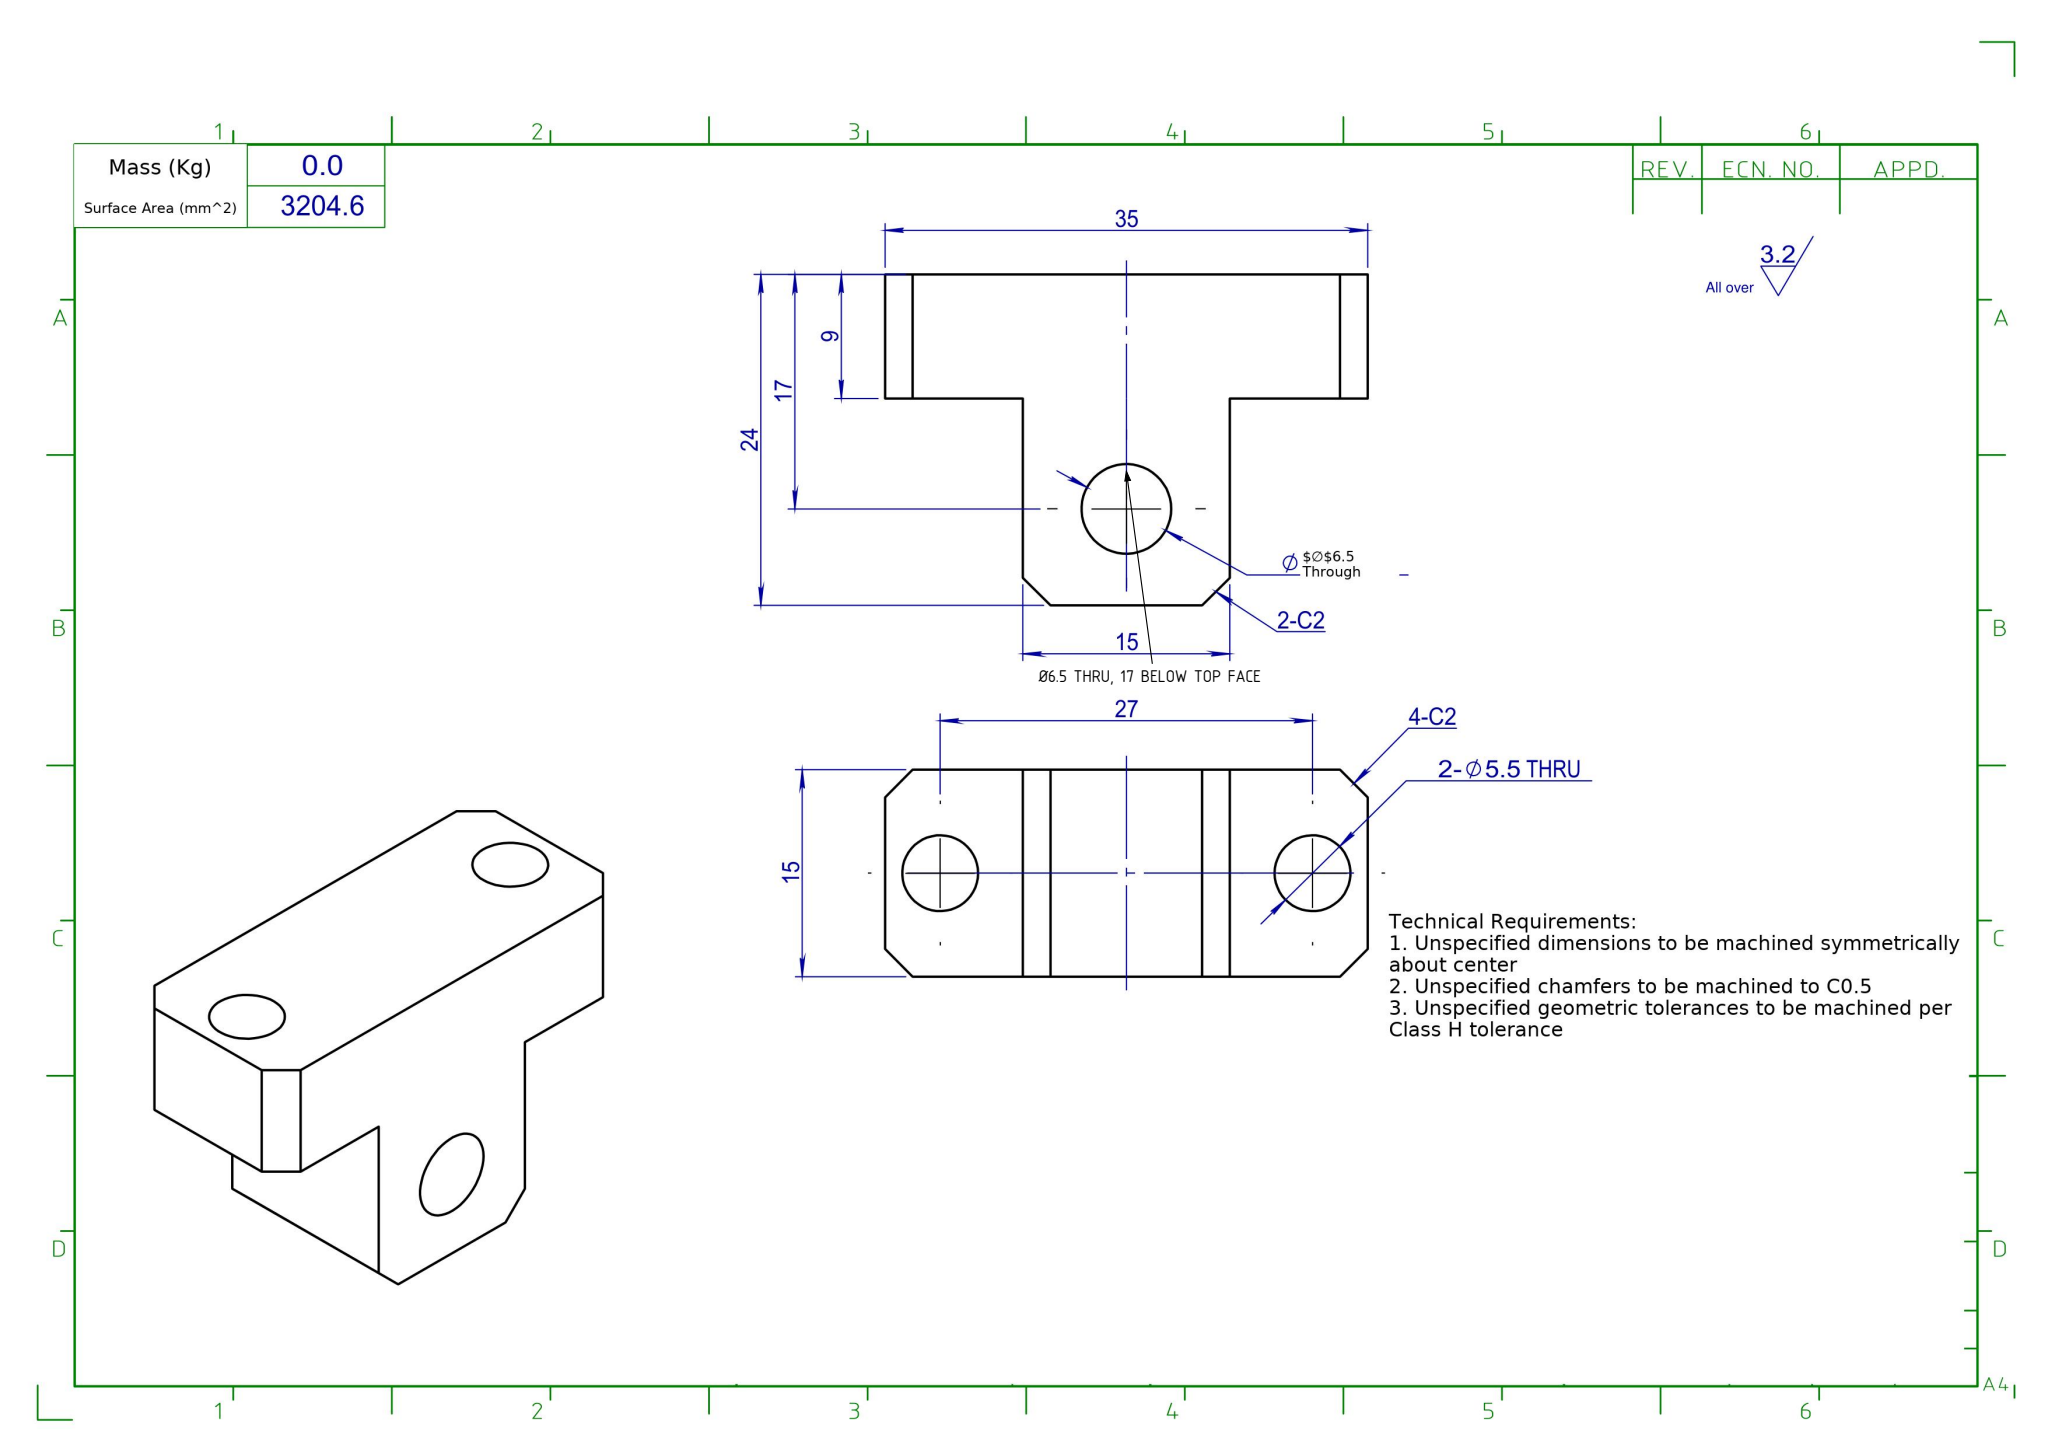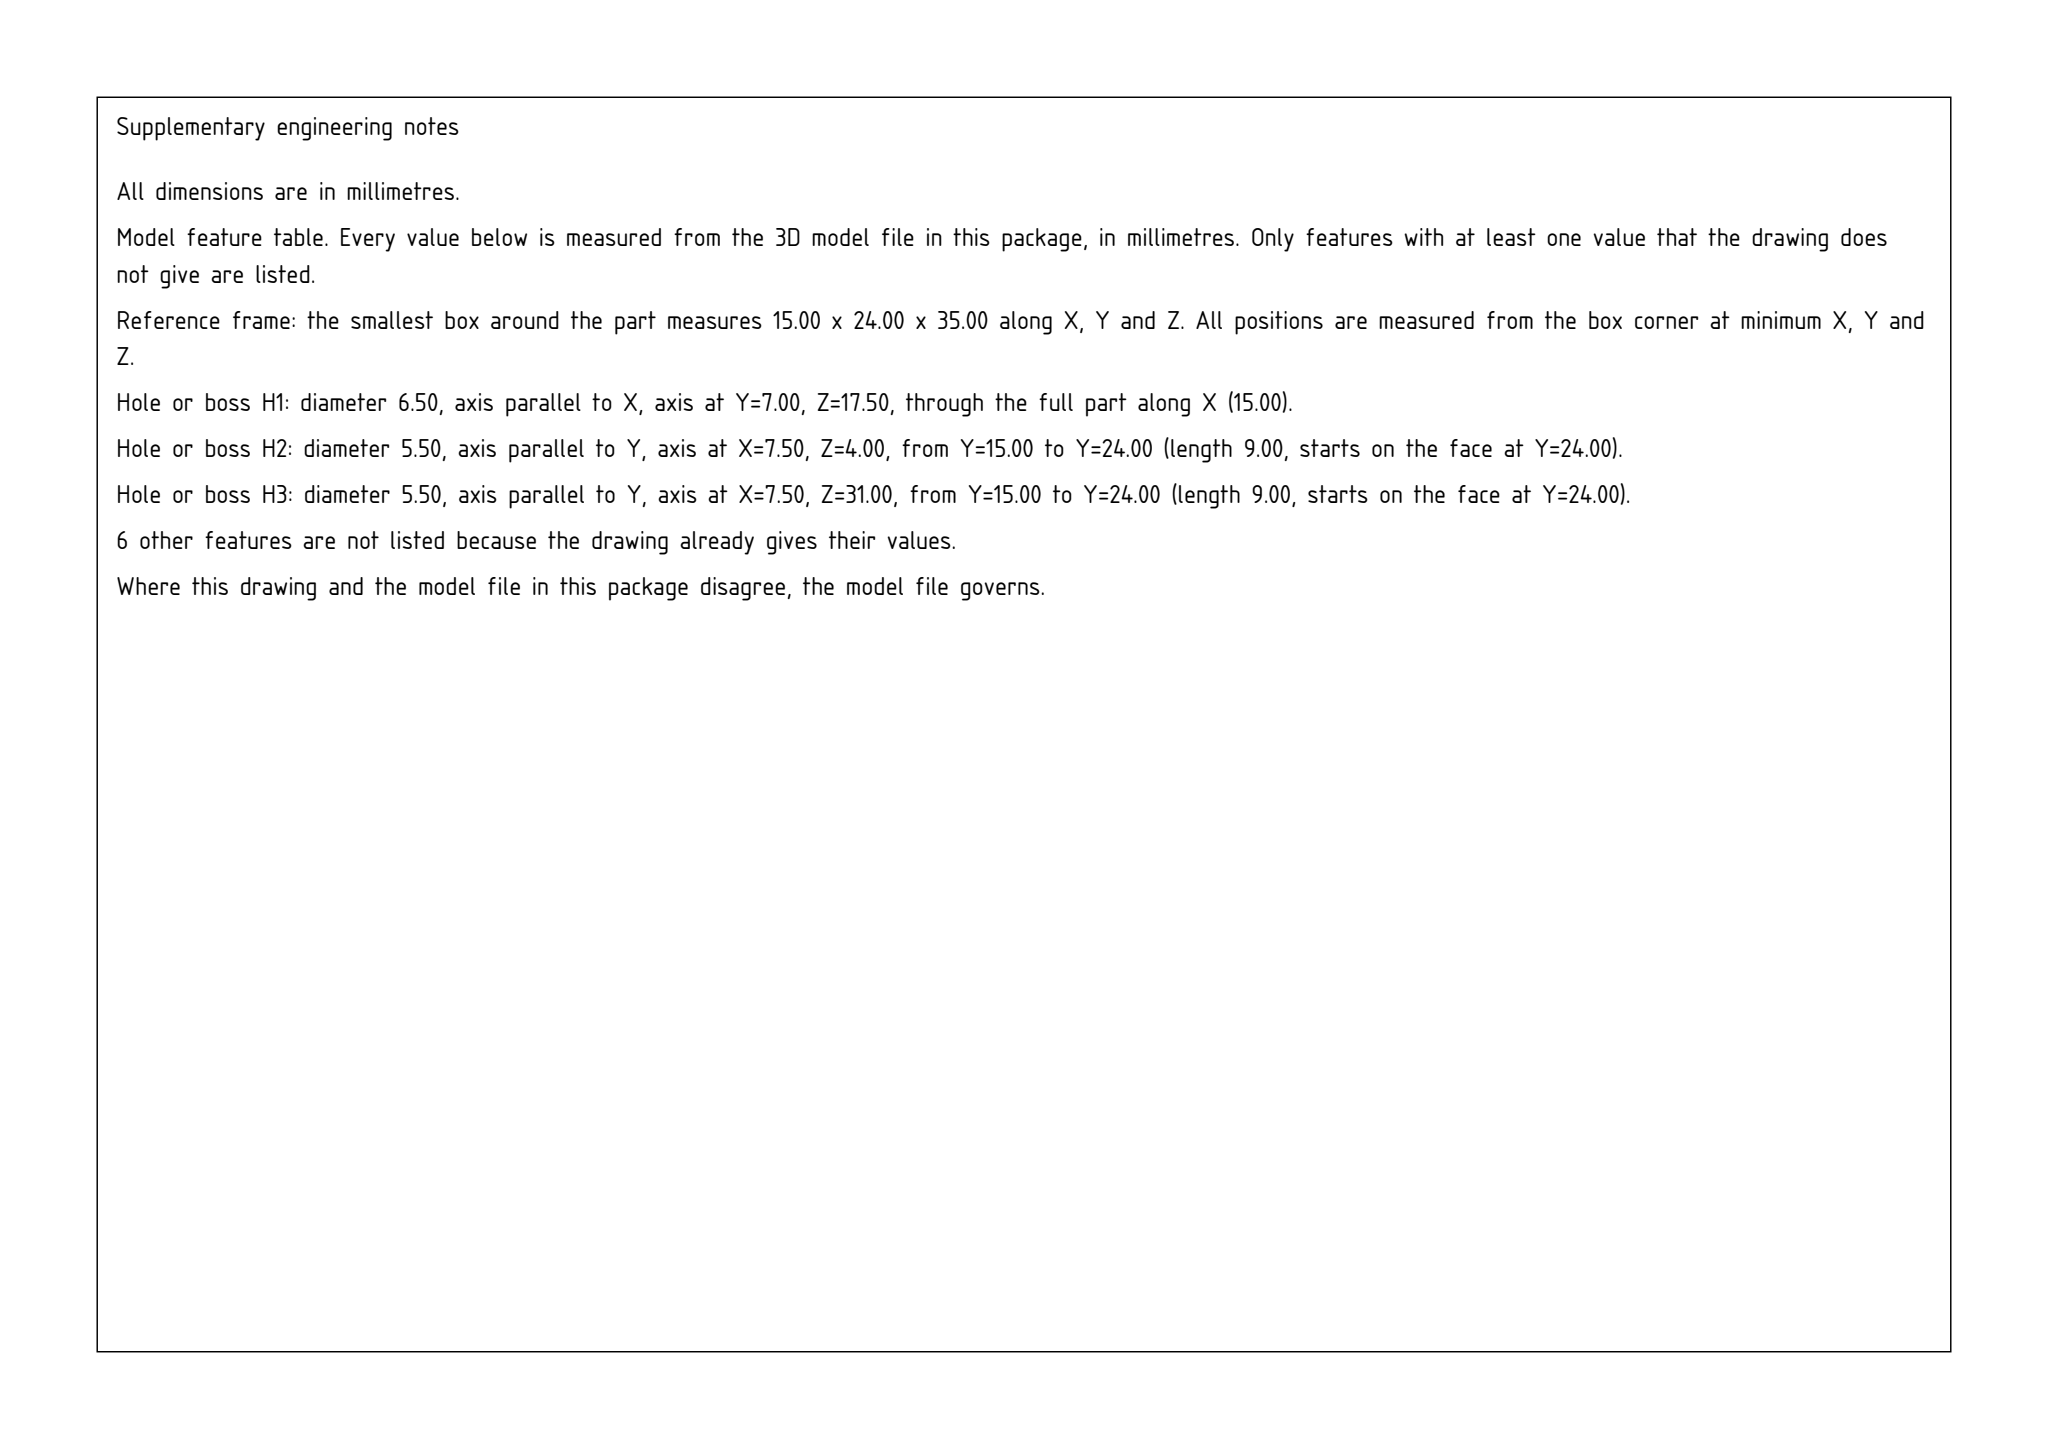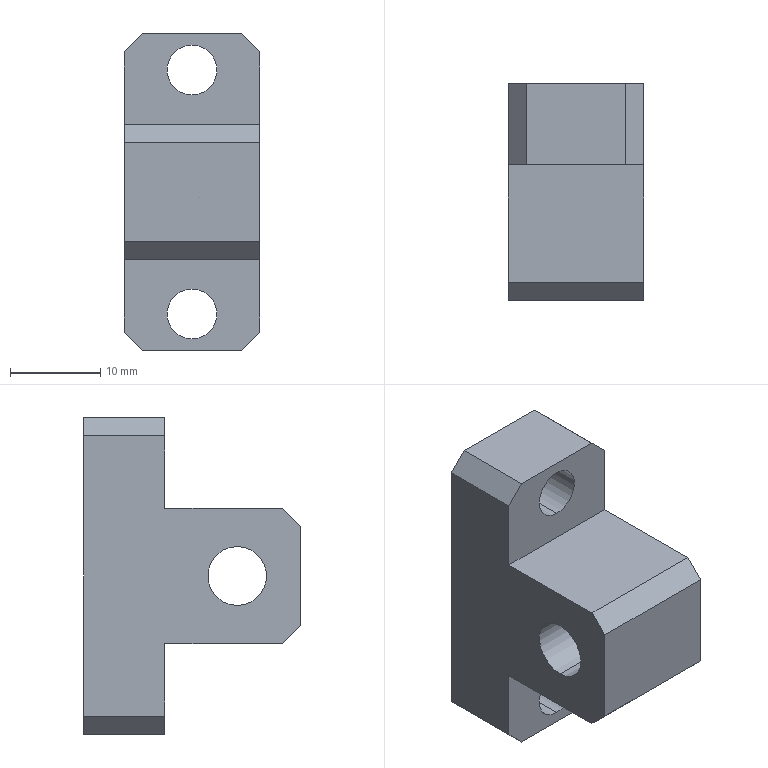Part | SolidWorks | mm | 1 solid | 22 faces | box 15 x 24 x 35 mm | volume 7043 mm3 | plane 16 | cylinder 6 | commonest cylinder face diameters 5.5 x4 6.5 x2
Drawing notes:
Ø6.5 THRU, CTR 17 BELOW TOP FACE, ON VERT CL | from the solid: cylinder hole/bore dia 6.5, axis x, from x=0 to 15 (thru), center y=7.0 of 24 height (=17 below top), z=17.5 = 35/2 centerline
build123d program:
from build123d import *

# Parameters (mm, degrees)
SKETCH1_W          = 15
SKETCH1_H          = 35
EXTRUDE1_DEPTH     = 24
SKETCH2_R          = 3.25
CUT_EXTRUDE1_DEPTH = 34.275
SKETCH3_W          = 15
SKETCH3_H          = 10
CUT_EXTRUDE2_DEPTH = 15
SKETCH4_R          = 2.75
CUT_EXTRUDE3_DEPTH = 25.238
CHAMFER1_SIZE      = 2


with BuildPart() as part:
    # Sketch1 → Extrude1 (new body)
    with BuildSketch(Plane(origin=(0, 0, 0), x_dir=(1, 0, 0), z_dir=(0, 1, 0))):
        Rectangle(SKETCH1_W, SKETCH1_H)
    extrude(amount=EXTRUDE1_DEPTH)

    # Sketch2 → Cut-Extrude1 (cut, through all)
    with BuildSketch(Plane(origin=(7.5, 0, 0), x_dir=(0, 0, -1), z_dir=(1, 0, 0))):
        with Locations((0, 7)):
            Circle(SKETCH2_R)
    extrude(amount=-CUT_EXTRUDE1_DEPTH, mode=Mode.SUBTRACT)

    # Sketch3 → Cut-Extrude2 (cut)
    with BuildSketch(Plane.XZ):
        with Locations((0, 12.5)):
            Rectangle(SKETCH3_W, SKETCH3_H)
        with Locations((0, -12.5)):
            Rectangle(SKETCH3_W, SKETCH3_H)
    extrude(amount=-CUT_EXTRUDE2_DEPTH, mode=Mode.SUBTRACT)

    # Sketch4 → Cut-Extrude3 (cut, through all)
    with BuildSketch(Plane.XZ.offset(-15)):
        with Locations(Location((0, 13.5, 0), (0, 0, 270))):
            Circle(SKETCH4_R)
        with Locations(Location((0, -13.5, 0), (0, 0, 90))):
            Circle(SKETCH4_R)
    extrude(amount=-CUT_EXTRUDE3_DEPTH, mode=Mode.SUBTRACT)

    # Chamfer1
    chamfer1_edges = [part.edges().sort_by_distance(p)[0] for p in [
        (0, 0, 7.5),
        (0, 0, -7.5),
        (-7.5, 19.5, -17.5),
        (7.5, 19.5, -17.5),
        (7.5, 19.5, 17.5),
        (-7.5, 19.5, 17.5),
    ]]
    chamfer(chamfer1_edges, length=CHAMFER1_SIZE)


solid = part.part
STEP:
#1=CARTESIAN_POINT('',(0.,24.,-10.75));
#2=VERTEX_POINT('',#1);
#3=CARTESIAN_POINT('',(0.,24.,-16.25));
#4=VERTEX_POINT('',#3);
#5=CARTESIAN_POINT('',(0.,24.,-13.5));
#6=DIRECTION('',(0.,-1.,0.));
#7=DIRECTION('',(0.,0.,1.));
#8=AXIS2_PLACEMENT_3D('',#5,#6,#7);
#9=CIRCLE('',#8,2.75);
#10=EDGE_CURVE('',#2,#4,#9,.T.);
#11=ORIENTED_EDGE('',*,*,#10,.F.);
#12=CARTESIAN_POINT('',(0.,15.,-10.75));
#13=VERTEX_POINT('',#12);
#14=CARTESIAN_POINT('',(0.,24.,-10.75));
#15=DIRECTION('',(0.,-1.,0.));
#16=VECTOR('',#15,1000.);
#17=LINE('',#14,#16);
#18=EDGE_CURVE('',#2,#13,#17,.T.);
#19=ORIENTED_EDGE('',*,*,#18,.T.);
#20=CARTESIAN_POINT('',(0.,15.,-16.25));
#21=VERTEX_POINT('',#20);
#22=CARTESIAN_POINT('',(0.,15.,-13.5));
#23=DIRECTION('',(0.,-1.,0.));
#24=DIRECTION('',(0.,0.,1.));
#25=AXIS2_PLACEMENT_3D('',#22,#23,#24);
#26=CIRCLE('',#25,2.75);
#27=EDGE_CURVE('',#13,#21,#26,.T.);
#28=ORIENTED_EDGE('',*,*,#27,.T.);
#29=CARTESIAN_POINT('',(0.,24.,-16.25));
#30=DIRECTION('',(0.,-1.,0.));
#31=VECTOR('',#30,1000.);
#32=LINE('',#29,#31);
#33=EDGE_CURVE('',#4,#21,#32,.T.);
#34=ORIENTED_EDGE('',*,*,#33,.F.);
#35=EDGE_LOOP('',(#11,#19,#28,#34));
#36=FACE_OUTER_BOUND('',#35,.T.);
#37=CARTESIAN_POINT('',(0.,24.,-13.5));
#38=DIRECTION('',(0.,-1.,0.));
#39=DIRECTION('',(0.,0.,-1.));
#40=AXIS2_PLACEMENT_3D('',#37,#38,#39);
#41=CYLINDRICAL_SURFACE('',#40,2.75);
#42=ADVANCED_FACE('',(#36),#41,.F.);
#43=CARTESIAN_POINT('',(0.,24.,16.25));
#44=VERTEX_POINT('',#43);
#45=CARTESIAN_POINT('',(0.,24.,10.75));
#46=VERTEX_POINT('',#45);
#47=CARTESIAN_POINT('',(0.,24.,13.5));
#48=DIRECTION('',(0.,-1.,0.));
#49=DIRECTION('',(0.,0.,-1.));
#50=AXIS2_PLACEMENT_3D('',#47,#48,#49);
#51=CIRCLE('',#50,2.75);
#52=EDGE_CURVE('',#44,#46,#51,.T.);
#53=ORIENTED_EDGE('',*,*,#52,.F.);
#54=CARTESIAN_POINT('',(0.,15.,16.25));
#55=VERTEX_POINT('',#54);
#56=CARTESIAN_POINT('',(0.,24.,16.25));
#57=DIRECTION('',(0.,-1.,0.));
#58=VECTOR('',#57,1000.);
#59=LINE('',#56,#58);
#60=EDGE_CURVE('',#44,#55,#59,.T.);
#61=ORIENTED_EDGE('',*,*,#60,.T.);
#62=CARTESIAN_POINT('',(0.,15.,10.75));
#63=VERTEX_POINT('',#62);
#64=CARTESIAN_POINT('',(0.,15.,13.5));
#65=DIRECTION('',(0.,-1.,0.));
#66=DIRECTION('',(0.,0.,-1.));
#67=AXIS2_PLACEMENT_3D('',#64,#65,#66);
#68=CIRCLE('',#67,2.75);
#69=EDGE_CURVE('',#55,#63,#68,.T.);
#70=ORIENTED_EDGE('',*,*,#69,.T.);
#71=CARTESIAN_POINT('',(0.,24.,10.75));
#72=DIRECTION('',(0.,-1.,0.));
#73=VECTOR('',#72,1000.);
#74=LINE('',#71,#73);
#75=EDGE_CURVE('',#46,#63,#74,.T.);
#76=ORIENTED_EDGE('',*,*,#75,.F.);
#77=EDGE_LOOP('',(#53,#61,#70,#76));
#78=FACE_OUTER_BOUND('',#77,.T.);
#79=CARTESIAN_POINT('',(0.,24.,13.5));
#80=DIRECTION('',(0.,-1.,0.));
#81=DIRECTION('',(0.,0.,-1.));
#82=AXIS2_PLACEMENT_3D('',#79,#80,#81);
#83=CYLINDRICAL_SURFACE('',#82,2.75);
#84=ADVANCED_FACE('',(#78),#83,.F.);
#85=CARTESIAN_POINT('',(-7.5,7.,3.25));
#86=VERTEX_POINT('',#85);
#87=CARTESIAN_POINT('',(-7.5,7.,-3.25));
#88=VERTEX_POINT('',#87);
#89=CARTESIAN_POINT('',(-7.5,7.,0.));
#90=DIRECTION('',(1.,0.,-0.));
#91=DIRECTION('',(0.,0.,-1.));
#92=AXIS2_PLACEMENT_3D('',#89,#90,#91);
#93=CIRCLE('',#92,3.25);
#94=EDGE_CURVE('',#86,#88,#93,.T.);
#95=ORIENTED_EDGE('',*,*,#94,.F.);
#96=CARTESIAN_POINT('',(7.5,7.,3.25));
#97=VERTEX_POINT('',#96);
#98=CARTESIAN_POINT('',(-7.5,7.,3.25));
#99=DIRECTION('',(1.,0.,-0.));
#100=VECTOR('',#99,1000.);
#101=LINE('',#98,#100);
#102=EDGE_CURVE('',#86,#97,#101,.T.);
#103=ORIENTED_EDGE('',*,*,#102,.T.);
#104=CARTESIAN_POINT('',(7.5,7.,-3.25));
#105=VERTEX_POINT('',#104);
#106=CARTESIAN_POINT('',(7.5,7.,-0.));
#107=DIRECTION('',(1.,0.,-0.));
#108=DIRECTION('',(0.,0.,-1.));
#109=AXIS2_PLACEMENT_3D('',#106,#107,#108);
#110=CIRCLE('',#109,3.25);
#111=EDGE_CURVE('',#97,#105,#110,.T.);
#112=ORIENTED_EDGE('',*,*,#111,.T.);
#113=CARTESIAN_POINT('',(-7.5,7.,-3.25));
#114=DIRECTION('',(1.,0.,-0.));
#115=VECTOR('',#114,1000.);
#116=LINE('',#113,#115);
#117=EDGE_CURVE('',#88,#105,#116,.T.);
#118=ORIENTED_EDGE('',*,*,#117,.F.);
#119=EDGE_LOOP('',(#95,#103,#112,#118));
#120=FACE_OUTER_BOUND('',#119,.T.);
#121=CARTESIAN_POINT('',(-7.5,7.,0.));
#122=DIRECTION('',(1.,0.,-0.));
#123=DIRECTION('',(0.,0.,-1.));
#124=AXIS2_PLACEMENT_3D('',#121,#122,#123);
#125=CYLINDRICAL_SURFACE('',#124,3.25);
#126=ADVANCED_FACE('',(#120),#125,.F.);
#127=CARTESIAN_POINT('',(5.5,24.,-17.5));
#128=VERTEX_POINT('',#127);
#129=CARTESIAN_POINT('',(-5.5,24.,-17.5));
#130=VERTEX_POINT('',#129);
#131=CARTESIAN_POINT('',(-7.5,24.,-17.5));
#132=DIRECTION('',(-1.,0.,0.));
#133=VECTOR('',#132,1000.);
#134=LINE('',#131,#133);
#135=EDGE_CURVE('',#128,#130,#134,.T.);
#136=ORIENTED_EDGE('',*,*,#135,.F.);
#137=CARTESIAN_POINT('',(5.5,15.,-17.5));
#138=VERTEX_POINT('',#137);
#139=CARTESIAN_POINT('',(5.5,24.,-17.5));
#140=DIRECTION('',(0.,-1.,0.));
#141=VECTOR('',#140,1000.);
#142=LINE('',#139,#141);
#143=EDGE_CURVE('',#128,#138,#142,.T.);
#144=ORIENTED_EDGE('',*,*,#143,.T.);
#145=CARTESIAN_POINT('',(-5.5,15.,-17.5));
#146=VERTEX_POINT('',#145);
#147=CARTESIAN_POINT('',(7.5,15.,-17.5));
#148=DIRECTION('',(1.,0.,0.));
#149=VECTOR('',#148,1000.);
#150=LINE('',#147,#149);
#151=EDGE_CURVE('',#146,#138,#150,.T.);
#152=ORIENTED_EDGE('',*,*,#151,.F.);
#153=CARTESIAN_POINT('',(-5.5,24.,-17.5));
#154=DIRECTION('',(0.,1.,0.));
#155=VECTOR('',#154,1000.);
#156=LINE('',#153,#155);
#157=EDGE_CURVE('',#146,#130,#156,.T.);
#158=ORIENTED_EDGE('',*,*,#157,.T.);
#159=EDGE_LOOP('',(#136,#144,#152,#158));
#160=FACE_OUTER_BOUND('',#159,.T.);
#161=CARTESIAN_POINT('',(-7.5,24.,-17.5));
#162=DIRECTION('',(0.,0.,1.));
#163=DIRECTION('',(1.,0.,0.));
#164=AXIS2_PLACEMENT_3D('',#161,#162,#163);
#165=PLANE('',#164);
#166=ADVANCED_FACE('',(#160),#165,.F.);
#167=CARTESIAN_POINT('',(5.5,15.,17.5));
#168=VERTEX_POINT('',#167);
#169=CARTESIAN_POINT('',(-5.5,15.,17.5));
#170=VERTEX_POINT('',#169);
#171=CARTESIAN_POINT('',(-7.5,15.,17.5));
#172=DIRECTION('',(-1.,0.,0.));
#173=VECTOR('',#172,1000.);
#174=LINE('',#171,#173);
#175=EDGE_CURVE('',#168,#170,#174,.T.);
#176=ORIENTED_EDGE('',*,*,#175,.F.);
#177=CARTESIAN_POINT('',(5.5,24.,17.5));
#178=VERTEX_POINT('',#177);
#179=CARTESIAN_POINT('',(5.5,24.,17.5));
#180=DIRECTION('',(0.,1.,0.));
#181=VECTOR('',#180,1000.);
#182=LINE('',#179,#181);
#183=EDGE_CURVE('',#168,#178,#182,.T.);
#184=ORIENTED_EDGE('',*,*,#183,.T.);
#185=CARTESIAN_POINT('',(-5.5,24.,17.5));
#186=VERTEX_POINT('',#185);
#187=CARTESIAN_POINT('',(-7.5,24.,17.5));
#188=DIRECTION('',(1.,0.,0.));
#189=VECTOR('',#188,1000.);
#190=LINE('',#187,#189);
#191=EDGE_CURVE('',#186,#178,#190,.T.);
#192=ORIENTED_EDGE('',*,*,#191,.F.);
#193=CARTESIAN_POINT('',(-5.5,24.,17.5));
#194=DIRECTION('',(0.,-1.,0.));
#195=VECTOR('',#194,1000.);
#196=LINE('',#193,#195);
#197=EDGE_CURVE('',#186,#170,#196,.T.);
#198=ORIENTED_EDGE('',*,*,#197,.T.);
#199=EDGE_LOOP('',(#176,#184,#192,#198));
#200=FACE_OUTER_BOUND('',#199,.T.);
#201=CARTESIAN_POINT('',(-7.5,24.,17.5));
#202=DIRECTION('',(0.,0.,-1.));
#203=DIRECTION('',(-1.,0.,0.));
#204=AXIS2_PLACEMENT_3D('',#201,#202,#203);
#205=PLANE('',#204);
#206=ADVANCED_FACE('',(#200),#205,.F.);
#207=CARTESIAN_POINT('',(-7.5,7.,0.));
#208=DIRECTION('',(1.,0.,-0.));
#209=DIRECTION('',(0.,0.,-1.));
#210=AXIS2_PLACEMENT_3D('',#207,#208,#209);
#211=CIRCLE('',#210,3.25);
#212=EDGE_CURVE('',#88,#86,#211,.T.);
#213=ORIENTED_EDGE('',*,*,#212,.T.);
#214=ORIENTED_EDGE('',*,*,#94,.T.);
#215=EDGE_LOOP('',(#213,#214));
#216=FACE_BOUND('',#215,.T.);
#217=CARTESIAN_POINT('',(-7.5,24.,-15.5));
#218=VERTEX_POINT('',#217);
#219=CARTESIAN_POINT('',(-7.5,24.,15.5));
#220=VERTEX_POINT('',#219);
#221=CARTESIAN_POINT('',(-7.5,24.,-17.5));
#222=DIRECTION('',(0.,0.,1.));
#223=VECTOR('',#222,1000.);
#224=LINE('',#221,#223);
#225=EDGE_CURVE('',#218,#220,#224,.T.);
#226=ORIENTED_EDGE('',*,*,#225,.F.);
#227=CARTESIAN_POINT('',(-7.5,15.,-15.5));
#228=VERTEX_POINT('',#227);
#229=CARTESIAN_POINT('',(-7.5,24.,-15.5));
#230=DIRECTION('',(0.,-1.,0.));
#231=VECTOR('',#230,1000.);
#232=LINE('',#229,#231);
#233=EDGE_CURVE('',#218,#228,#232,.T.);
#234=ORIENTED_EDGE('',*,*,#233,.T.);
#235=CARTESIAN_POINT('',(-7.5,15.,-7.5));
#236=VERTEX_POINT('',#235);
#237=CARTESIAN_POINT('',(-7.5,15.,-17.5));
#238=DIRECTION('',(-0.,0.,-1.));
#239=VECTOR('',#238,1000.);
#240=LINE('',#237,#239);
#241=EDGE_CURVE('',#236,#228,#240,.T.);
#242=ORIENTED_EDGE('',*,*,#241,.F.);
#243=CARTESIAN_POINT('',(-7.5,2.,-7.5));
#244=VERTEX_POINT('',#243);
#245=CARTESIAN_POINT('',(-7.5,15.,-7.5));
#246=DIRECTION('',(0.,-1.,0.));
#247=VECTOR('',#246,1000.);
#248=LINE('',#245,#247);
#249=EDGE_CURVE('',#236,#244,#248,.T.);
#250=ORIENTED_EDGE('',*,*,#249,.T.);
#251=CARTESIAN_POINT('',(-7.5,0.,-5.5));
#252=VERTEX_POINT('',#251);
#253=CARTESIAN_POINT('',(-7.5,2.,-7.5));
#254=DIRECTION('',(0.,-0.7071,0.7071));
#255=VECTOR('',#254,1000.);
#256=LINE('',#253,#255);
#257=EDGE_CURVE('',#244,#252,#256,.T.);
#258=ORIENTED_EDGE('',*,*,#257,.T.);
#259=CARTESIAN_POINT('',(-7.5,-0.,5.5));
#260=VERTEX_POINT('',#259);
#261=CARTESIAN_POINT('',(-7.5,0.,-17.5));
#262=DIRECTION('',(0.,0.,1.));
#263=VECTOR('',#262,1000.);
#264=LINE('',#261,#263);
#265=EDGE_CURVE('',#252,#260,#264,.T.);
#266=ORIENTED_EDGE('',*,*,#265,.T.);
#267=CARTESIAN_POINT('',(-7.5,2.,7.5));
#268=VERTEX_POINT('',#267);
#269=CARTESIAN_POINT('',(-7.5,2.,7.5));
#270=DIRECTION('',(0.,0.7071,0.7071));
#271=VECTOR('',#270,1000.);
#272=LINE('',#269,#271);
#273=EDGE_CURVE('',#260,#268,#272,.T.);
#274=ORIENTED_EDGE('',*,*,#273,.T.);
#275=CARTESIAN_POINT('',(-7.5,15.,7.5));
#276=VERTEX_POINT('',#275);
#277=CARTESIAN_POINT('',(-7.5,15.,7.5));
#278=DIRECTION('',(0.,-1.,0.));
#279=VECTOR('',#278,1000.);
#280=LINE('',#277,#279);
#281=EDGE_CURVE('',#276,#268,#280,.T.);
#282=ORIENTED_EDGE('',*,*,#281,.F.);
#283=CARTESIAN_POINT('',(-7.5,15.,15.5));
#284=VERTEX_POINT('',#283);
#285=CARTESIAN_POINT('',(-7.5,15.,17.5));
#286=DIRECTION('',(0.,0.,-1.));
#287=VECTOR('',#286,1000.);
#288=LINE('',#285,#287);
#289=EDGE_CURVE('',#284,#276,#288,.T.);
#290=ORIENTED_EDGE('',*,*,#289,.F.);
#291=CARTESIAN_POINT('',(-7.5,24.,15.5));
#292=DIRECTION('',(0.,1.,0.));
#293=VECTOR('',#292,1000.);
#294=LINE('',#291,#293);
#295=EDGE_CURVE('',#284,#220,#294,.T.);
#296=ORIENTED_EDGE('',*,*,#295,.T.);
#297=EDGE_LOOP('',(#226,#234,#242,#250,#258,#266,#274,#282,#290,#296));
#298=FACE_OUTER_BOUND('',#297,.T.);
#299=CARTESIAN_POINT('',(-7.5,24.,-17.5));
#300=DIRECTION('',(1.,0.,-0.));
#301=DIRECTION('',(-0.,0.,-1.));
#302=AXIS2_PLACEMENT_3D('',#299,#300,#301);
#303=PLANE('',#302);
#304=ADVANCED_FACE('',(#216,#298),#303,.F.);
#305=CARTESIAN_POINT('',(7.5,7.,-0.));
#306=DIRECTION('',(1.,0.,-0.));
#307=DIRECTION('',(0.,0.,-1.));
#308=AXIS2_PLACEMENT_3D('',#305,#306,#307);
#309=CIRCLE('',#308,3.25);
#310=EDGE_CURVE('',#105,#97,#309,.T.);
#311=ORIENTED_EDGE('',*,*,#310,.F.);
#312=ORIENTED_EDGE('',*,*,#111,.F.);
#313=EDGE_LOOP('',(#311,#312));
#314=FACE_BOUND('',#313,.T.);
#315=CARTESIAN_POINT('',(7.5,15.,-15.5));
#316=VERTEX_POINT('',#315);
#317=CARTESIAN_POINT('',(7.5,15.,-7.5));
#318=VERTEX_POINT('',#317);
#319=CARTESIAN_POINT('',(7.5,15.,-17.5));
#320=DIRECTION('',(0.,0.,1.));
#321=VECTOR('',#320,1000.);
#322=LINE('',#319,#321);
#323=EDGE_CURVE('',#316,#318,#322,.T.);
#324=ORIENTED_EDGE('',*,*,#323,.F.);
#325=CARTESIAN_POINT('',(7.5,24.,-15.5));
#326=VERTEX_POINT('',#325);
#327=CARTESIAN_POINT('',(7.5,24.,-15.5));
#328=DIRECTION('',(0.,1.,0.));
#329=VECTOR('',#328,1000.);
#330=LINE('',#327,#329);
#331=EDGE_CURVE('',#316,#326,#330,.T.);
#332=ORIENTED_EDGE('',*,*,#331,.T.);
#333=CARTESIAN_POINT('',(7.5,24.,15.5));
#334=VERTEX_POINT('',#333);
#335=CARTESIAN_POINT('',(7.5,24.,-17.5));
#336=DIRECTION('',(-0.,0.,-1.));
#337=VECTOR('',#336,1000.);
#338=LINE('',#335,#337);
#339=EDGE_CURVE('',#334,#326,#338,.T.);
#340=ORIENTED_EDGE('',*,*,#339,.F.);
#341=CARTESIAN_POINT('',(7.5,15.,15.5));
#342=VERTEX_POINT('',#341);
#343=CARTESIAN_POINT('',(7.5,24.,15.5));
#344=DIRECTION('',(0.,-1.,0.));
#345=VECTOR('',#344,1000.);
#346=LINE('',#343,#345);
#347=EDGE_CURVE('',#334,#342,#346,.T.);
#348=ORIENTED_EDGE('',*,*,#347,.T.);
#349=CARTESIAN_POINT('',(7.5,15.,7.5));
#350=VERTEX_POINT('',#349);
#351=CARTESIAN_POINT('',(7.5,15.,17.5));
#352=DIRECTION('',(-0.,0.,1.));
#353=VECTOR('',#352,1000.);
#354=LINE('',#351,#353);
#355=EDGE_CURVE('',#350,#342,#354,.T.);
#356=ORIENTED_EDGE('',*,*,#355,.F.);
#357=CARTESIAN_POINT('',(7.5,2.,7.5));
#358=VERTEX_POINT('',#357);
#359=CARTESIAN_POINT('',(7.5,15.,7.5));
#360=DIRECTION('',(0.,-1.,0.));
#361=VECTOR('',#360,1000.);
#362=LINE('',#359,#361);
#363=EDGE_CURVE('',#350,#358,#362,.T.);
#364=ORIENTED_EDGE('',*,*,#363,.T.);
#365=CARTESIAN_POINT('',(7.5,0.,5.5));
#366=VERTEX_POINT('',#365);
#367=CARTESIAN_POINT('',(7.5,2.,7.5));
#368=DIRECTION('',(-0.,-0.7071,-0.7071));
#369=VECTOR('',#368,1000.);
#370=LINE('',#367,#369);
#371=EDGE_CURVE('',#358,#366,#370,.T.);
#372=ORIENTED_EDGE('',*,*,#371,.T.);
#373=CARTESIAN_POINT('',(7.5,0.,-5.5));
#374=VERTEX_POINT('',#373);
#375=CARTESIAN_POINT('',(7.5,0.,-17.5));
#376=DIRECTION('',(-0.,0.,-1.));
#377=VECTOR('',#376,1000.);
#378=LINE('',#375,#377);
#379=EDGE_CURVE('',#366,#374,#378,.T.);
#380=ORIENTED_EDGE('',*,*,#379,.T.);
#381=CARTESIAN_POINT('',(7.5,2.,-7.5));
#382=VERTEX_POINT('',#381);
#383=CARTESIAN_POINT('',(7.5,2.,-7.5));
#384=DIRECTION('',(-0.,0.7071,-0.7071));
#385=VECTOR('',#384,1000.);
#386=LINE('',#383,#385);
#387=EDGE_CURVE('',#374,#382,#386,.T.);
#388=ORIENTED_EDGE('',*,*,#387,.T.);
#389=CARTESIAN_POINT('',(7.5,15.,-7.5));
#390=DIRECTION('',(0.,-1.,0.));
#391=VECTOR('',#390,1000.);
#392=LINE('',#389,#391);
#393=EDGE_CURVE('',#318,#382,#392,.T.);
#394=ORIENTED_EDGE('',*,*,#393,.F.);
#395=EDGE_LOOP('',(#324,#332,#340,#348,#356,#364,#372,#380,#388,#394));
#396=FACE_OUTER_BOUND('',#395,.T.);
#397=CARTESIAN_POINT('',(7.5,24.,-17.5));
#398=DIRECTION('',(-1.,0.,0.));
#399=DIRECTION('',(0.,0.,1.));
#400=AXIS2_PLACEMENT_3D('',#397,#398,#399);
#401=PLANE('',#400);
#402=ADVANCED_FACE('',(#314,#396),#401,.F.);
#403=CARTESIAN_POINT('',(0.,24.,-13.5));
#404=DIRECTION('',(0.,-1.,0.));
#405=DIRECTION('',(0.,0.,1.));
#406=AXIS2_PLACEMENT_3D('',#403,#404,#405);
#407=CIRCLE('',#406,2.75);
#408=EDGE_CURVE('',#4,#2,#407,.T.);
#409=ORIENTED_EDGE('',*,*,#408,.T.);
#410=ORIENTED_EDGE('',*,*,#10,.T.);
#411=EDGE_LOOP('',(#409,#410));
#412=FACE_BOUND('',#411,.T.);
#413=CARTESIAN_POINT('',(0.,24.,13.5));
#414=DIRECTION('',(0.,-1.,0.));
#415=DIRECTION('',(0.,0.,-1.));
#416=AXIS2_PLACEMENT_3D('',#413,#414,#415);
#417=CIRCLE('',#416,2.75);
#418=EDGE_CURVE('',#46,#44,#417,.T.);
#419=ORIENTED_EDGE('',*,*,#418,.T.);
#420=ORIENTED_EDGE('',*,*,#52,.T.);
#421=EDGE_LOOP('',(#419,#420));
#422=FACE_BOUND('',#421,.T.);
#423=ORIENTED_EDGE('',*,*,#339,.T.);
#424=CARTESIAN_POINT('',(16.5,24.,-6.5));
#425=DIRECTION('',(-0.7071,0.,-0.7071));
#426=VECTOR('',#425,1000.);
#427=LINE('',#424,#426);
#428=EDGE_CURVE('',#326,#128,#427,.T.);
#429=ORIENTED_EDGE('',*,*,#428,.T.);
#430=ORIENTED_EDGE('',*,*,#135,.T.);
#431=CARTESIAN_POINT('',(-24.,24.,1.));
#432=DIRECTION('',(-0.7071,0.,0.7071));
#433=VECTOR('',#432,1000.);
#434=LINE('',#431,#433);
#435=EDGE_CURVE('',#130,#218,#434,.T.);
#436=ORIENTED_EDGE('',*,*,#435,.T.);
#437=ORIENTED_EDGE('',*,*,#225,.T.);
#438=CARTESIAN_POINT('',(-6.5,24.,16.5));
#439=DIRECTION('',(0.7071,0.,0.7071));
#440=VECTOR('',#439,1000.);
#441=LINE('',#438,#440);
#442=EDGE_CURVE('',#220,#186,#441,.T.);
#443=ORIENTED_EDGE('',*,*,#442,.T.);
#444=ORIENTED_EDGE('',*,*,#191,.T.);
#445=CARTESIAN_POINT('',(-1.,24.,24.));
#446=DIRECTION('',(0.7071,0.,-0.7071));
#447=VECTOR('',#446,1000.);
#448=LINE('',#445,#447);
#449=EDGE_CURVE('',#178,#334,#448,.T.);
#450=ORIENTED_EDGE('',*,*,#449,.T.);
#451=EDGE_LOOP('',(#423,#429,#430,#436,#437,#443,#444,#450));
#452=FACE_OUTER_BOUND('',#451,.T.);
#453=CARTESIAN_POINT('',(-7.5,24.,17.5));
#454=DIRECTION('',(0.,1.,0.));
#455=DIRECTION('',(0.,0.,1.));
#456=AXIS2_PLACEMENT_3D('',#453,#454,#455);
#457=PLANE('',#456);
#458=ADVANCED_FACE('',(#412,#422,#452),#457,.T.);
#459=ORIENTED_EDGE('',*,*,#265,.F.);
#460=CARTESIAN_POINT('',(-7.5,0.,-5.5));
#461=DIRECTION('',(1.,0.,0.));
#462=VECTOR('',#461,1000.);
#463=LINE('',#460,#462);
#464=EDGE_CURVE('',#252,#374,#463,.T.);
#465=ORIENTED_EDGE('',*,*,#464,.T.);
#466=ORIENTED_EDGE('',*,*,#379,.F.);
#467=CARTESIAN_POINT('',(-7.5,0.,5.5));
#468=DIRECTION('',(-1.,0.,0.));
#469=VECTOR('',#468,1000.);
#470=LINE('',#467,#469);
#471=EDGE_CURVE('',#366,#260,#470,.T.);
#472=ORIENTED_EDGE('',*,*,#471,.T.);
#473=EDGE_LOOP('',(#459,#465,#466,#472));
#474=FACE_OUTER_BOUND('',#473,.T.);
#475=CARTESIAN_POINT('',(-7.5,0.,17.5));
#476=DIRECTION('',(0.,1.,0.));
#477=DIRECTION('',(0.,0.,1.));
#478=AXIS2_PLACEMENT_3D('',#475,#476,#477);
#479=PLANE('',#478);
#480=ADVANCED_FACE('',(#474),#479,.F.);
#481=ORIENTED_EDGE('',*,*,#102,.F.);
#482=ORIENTED_EDGE('',*,*,#212,.F.);
#483=ORIENTED_EDGE('',*,*,#117,.T.);
#484=ORIENTED_EDGE('',*,*,#310,.T.);
#485=EDGE_LOOP('',(#481,#482,#483,#484));
#486=FACE_OUTER_BOUND('',#485,.T.);
#487=CARTESIAN_POINT('',(-7.5,7.,0.));
#488=DIRECTION('',(1.,0.,-0.));
#489=DIRECTION('',(0.,0.,-1.));
#490=AXIS2_PLACEMENT_3D('',#487,#488,#489);
#491=CYLINDRICAL_SURFACE('',#490,3.25);
#492=ADVANCED_FACE('',(#486),#491,.F.);
#493=ORIENTED_EDGE('',*,*,#281,.T.);
#494=CARTESIAN_POINT('',(-7.5,2.,7.5));
#495=DIRECTION('',(1.,0.,0.));
#496=VECTOR('',#495,1000.);
#497=LINE('',#494,#496);
#498=EDGE_CURVE('',#268,#358,#497,.T.);
#499=ORIENTED_EDGE('',*,*,#498,.T.);
#500=ORIENTED_EDGE('',*,*,#363,.F.);
#501=CARTESIAN_POINT('',(-7.5,15.,7.5));
#502=DIRECTION('',(1.,0.,0.));
#503=VECTOR('',#502,1000.);
#504=LINE('',#501,#503);
#505=EDGE_CURVE('',#276,#350,#504,.T.);
#506=ORIENTED_EDGE('',*,*,#505,.F.);
#507=EDGE_LOOP('',(#493,#499,#500,#506));
#508=FACE_OUTER_BOUND('',#507,.T.);
#509=CARTESIAN_POINT('',(-7.5,15.,7.5));
#510=DIRECTION('',(0.,0.,-1.));
#511=DIRECTION('',(-1.,0.,0.));
#512=AXIS2_PLACEMENT_3D('',#509,#510,#511);
#513=PLANE('',#512);
#514=ADVANCED_FACE('',(#508),#513,.F.);
#515=CARTESIAN_POINT('',(0.,15.,13.5));
#516=DIRECTION('',(0.,-1.,0.));
#517=DIRECTION('',(0.,0.,-1.));
#518=AXIS2_PLACEMENT_3D('',#515,#516,#517);
#519=CIRCLE('',#518,2.75);
#520=EDGE_CURVE('',#63,#55,#519,.T.);
#521=ORIENTED_EDGE('',*,*,#520,.F.);
#522=ORIENTED_EDGE('',*,*,#69,.F.);
#523=EDGE_LOOP('',(#521,#522));
#524=FACE_BOUND('',#523,.T.);
#525=ORIENTED_EDGE('',*,*,#355,.T.);
#526=CARTESIAN_POINT('',(4.,15.,19.));
#527=DIRECTION('',(-0.7071,0.,0.7071));
#528=VECTOR('',#527,1000.);
#529=LINE('',#526,#528);
#530=EDGE_CURVE('',#342,#168,#529,.T.);
#531=ORIENTED_EDGE('',*,*,#530,.T.);
#532=ORIENTED_EDGE('',*,*,#175,.T.);
#533=CARTESIAN_POINT('',(-11.5,15.,11.5));
#534=DIRECTION('',(-0.7071,0.,-0.7071));
#535=VECTOR('',#534,1000.);
#536=LINE('',#533,#535);
#537=EDGE_CURVE('',#170,#284,#536,.T.);
#538=ORIENTED_EDGE('',*,*,#537,.T.);
#539=ORIENTED_EDGE('',*,*,#289,.T.);
#540=ORIENTED_EDGE('',*,*,#505,.T.);
#541=EDGE_LOOP('',(#525,#531,#532,#538,#539,#540));
#542=FACE_OUTER_BOUND('',#541,.T.);
#543=CARTESIAN_POINT('',(-7.5,15.,7.5));
#544=DIRECTION('',(0.,-1.,0.));
#545=DIRECTION('',(0.,0.,-1.));
#546=AXIS2_PLACEMENT_3D('',#543,#544,#545);
#547=PLANE('',#546);
#548=ADVANCED_FACE('',(#524,#542),#547,.T.);
#549=ORIENTED_EDGE('',*,*,#393,.T.);
#550=CARTESIAN_POINT('',(7.5,2.,-7.5));
#551=DIRECTION('',(-1.,0.,0.));
#552=VECTOR('',#551,1000.);
#553=LINE('',#550,#552);
#554=EDGE_CURVE('',#382,#244,#553,.T.);
#555=ORIENTED_EDGE('',*,*,#554,.T.);
#556=ORIENTED_EDGE('',*,*,#249,.F.);
#557=CARTESIAN_POINT('',(7.5,15.,-7.5));
#558=DIRECTION('',(-1.,0.,0.));
#559=VECTOR('',#558,1000.);
#560=LINE('',#557,#559);
#561=EDGE_CURVE('',#318,#236,#560,.T.);
#562=ORIENTED_EDGE('',*,*,#561,.F.);
#563=EDGE_LOOP('',(#549,#555,#556,#562));
#564=FACE_OUTER_BOUND('',#563,.T.);
#565=CARTESIAN_POINT('',(7.5,15.,-7.5));
#566=DIRECTION('',(0.,0.,1.));
#567=DIRECTION('',(1.,0.,0.));
#568=AXIS2_PLACEMENT_3D('',#565,#566,#567);
#569=PLANE('',#568);
#570=ADVANCED_FACE('',(#564),#569,.F.);
#571=CARTESIAN_POINT('',(0.,15.,-13.5));
#572=DIRECTION('',(0.,-1.,0.));
#573=DIRECTION('',(0.,0.,1.));
#574=AXIS2_PLACEMENT_3D('',#571,#572,#573);
#575=CIRCLE('',#574,2.75);
#576=EDGE_CURVE('',#21,#13,#575,.T.);
#577=ORIENTED_EDGE('',*,*,#576,.F.);
#578=ORIENTED_EDGE('',*,*,#27,.F.);
#579=EDGE_LOOP('',(#577,#578));
#580=FACE_BOUND('',#579,.T.);
#581=ORIENTED_EDGE('',*,*,#151,.T.);
#582=CARTESIAN_POINT('',(11.5,15.,-11.5));
#583=DIRECTION('',(0.7071,0.,0.7071));
#584=VECTOR('',#583,1000.);
#585=LINE('',#582,#584);
#586=EDGE_CURVE('',#138,#316,#585,.T.);
#587=ORIENTED_EDGE('',*,*,#586,.T.);
#588=ORIENTED_EDGE('',*,*,#323,.T.);
#589=ORIENTED_EDGE('',*,*,#561,.T.);
#590=ORIENTED_EDGE('',*,*,#241,.T.);
#591=CARTESIAN_POINT('',(-4.,15.,-19.));
#592=DIRECTION('',(0.7071,0.,-0.7071));
#593=VECTOR('',#592,1000.);
#594=LINE('',#591,#593);
#595=EDGE_CURVE('',#228,#146,#594,.T.);
#596=ORIENTED_EDGE('',*,*,#595,.T.);
#597=EDGE_LOOP('',(#581,#587,#588,#589,#590,#596));
#598=FACE_OUTER_BOUND('',#597,.T.);
#599=CARTESIAN_POINT('',(7.5,15.,-7.5));
#600=DIRECTION('',(0.,-1.,0.));
#601=DIRECTION('',(0.,0.,-1.));
#602=AXIS2_PLACEMENT_3D('',#599,#600,#601);
#603=PLANE('',#602);
#604=ADVANCED_FACE('',(#580,#598),#603,.T.);
#605=ORIENTED_EDGE('',*,*,#60,.F.);
#606=ORIENTED_EDGE('',*,*,#418,.F.);
#607=ORIENTED_EDGE('',*,*,#75,.T.);
#608=ORIENTED_EDGE('',*,*,#520,.T.);
#609=EDGE_LOOP('',(#605,#606,#607,#608));
#610=FACE_OUTER_BOUND('',#609,.T.);
#611=CARTESIAN_POINT('',(0.,24.,13.5));
#612=DIRECTION('',(0.,-1.,0.));
#613=DIRECTION('',(0.,0.,-1.));
#614=AXIS2_PLACEMENT_3D('',#611,#612,#613);
#615=CYLINDRICAL_SURFACE('',#614,2.75);
#616=ADVANCED_FACE('',(#610),#615,.F.);
#617=ORIENTED_EDGE('',*,*,#18,.F.);
#618=ORIENTED_EDGE('',*,*,#408,.F.);
#619=ORIENTED_EDGE('',*,*,#33,.T.);
#620=ORIENTED_EDGE('',*,*,#576,.T.);
#621=EDGE_LOOP('',(#617,#618,#619,#620));
#622=FACE_OUTER_BOUND('',#621,.T.);
#623=CARTESIAN_POINT('',(0.,24.,-13.5));
#624=DIRECTION('',(0.,-1.,0.));
#625=DIRECTION('',(0.,0.,-1.));
#626=AXIS2_PLACEMENT_3D('',#623,#624,#625);
#627=CYLINDRICAL_SURFACE('',#626,2.75);
#628=ADVANCED_FACE('',(#622),#627,.F.);
#629=ORIENTED_EDGE('',*,*,#428,.F.);
#630=ORIENTED_EDGE('',*,*,#331,.F.);
#631=ORIENTED_EDGE('',*,*,#586,.F.);
#632=ORIENTED_EDGE('',*,*,#143,.F.);
#633=EDGE_LOOP('',(#629,#630,#631,#632));
#634=FACE_OUTER_BOUND('',#633,.T.);
#635=CARTESIAN_POINT('',(5.5,24.,-17.5));
#636=DIRECTION('',(-0.7071,0.,0.7071));
#637=DIRECTION('',(0.,-1.,0.));
#638=AXIS2_PLACEMENT_3D('',#635,#636,#637);
#639=PLANE('',#638);
#640=ADVANCED_FACE('',(#634),#639,.F.);
#641=ORIENTED_EDGE('',*,*,#435,.F.);
#642=ORIENTED_EDGE('',*,*,#157,.F.);
#643=ORIENTED_EDGE('',*,*,#595,.F.);
#644=ORIENTED_EDGE('',*,*,#233,.F.);
#645=EDGE_LOOP('',(#641,#642,#643,#644));
#646=FACE_OUTER_BOUND('',#645,.T.);
#647=CARTESIAN_POINT('',(-7.5,24.,-15.5));
#648=DIRECTION('',(0.7071,0.,0.7071));
#649=DIRECTION('',(0.,-1.,0.));
#650=AXIS2_PLACEMENT_3D('',#647,#648,#649);
#651=PLANE('',#650);
#652=ADVANCED_FACE('',(#646),#651,.F.);
#653=ORIENTED_EDGE('',*,*,#387,.F.);
#654=ORIENTED_EDGE('',*,*,#464,.F.);
#655=ORIENTED_EDGE('',*,*,#257,.F.);
#656=ORIENTED_EDGE('',*,*,#554,.F.);
#657=EDGE_LOOP('',(#653,#654,#655,#656));
#658=FACE_OUTER_BOUND('',#657,.T.);
#659=CARTESIAN_POINT('',(7.5,2.,-7.5));
#660=DIRECTION('',(0.,0.7071,0.7071));
#661=DIRECTION('',(-1.,0.,0.));
#662=AXIS2_PLACEMENT_3D('',#659,#660,#661);
#663=PLANE('',#662);
#664=ADVANCED_FACE('',(#658),#663,.F.);
#665=ORIENTED_EDGE('',*,*,#273,.F.);
#666=ORIENTED_EDGE('',*,*,#471,.F.);
#667=ORIENTED_EDGE('',*,*,#371,.F.);
#668=ORIENTED_EDGE('',*,*,#498,.F.);
#669=EDGE_LOOP('',(#665,#666,#667,#668));
#670=FACE_OUTER_BOUND('',#669,.T.);
#671=CARTESIAN_POINT('',(-7.5,2.,7.5));
#672=DIRECTION('',(0.,0.7071,-0.7071));
#673=DIRECTION('',(1.,0.,0.));
#674=AXIS2_PLACEMENT_3D('',#671,#672,#673);
#675=PLANE('',#674);
#676=ADVANCED_FACE('',(#670),#675,.F.);
#677=ORIENTED_EDGE('',*,*,#449,.F.);
#678=ORIENTED_EDGE('',*,*,#183,.F.);
#679=ORIENTED_EDGE('',*,*,#530,.F.);
#680=ORIENTED_EDGE('',*,*,#347,.F.);
#681=EDGE_LOOP('',(#677,#678,#679,#680));
#682=FACE_OUTER_BOUND('',#681,.T.);
#683=CARTESIAN_POINT('',(7.5,24.,15.5));
#684=DIRECTION('',(-0.7071,0.,-0.7071));
#685=DIRECTION('',(0.,-1.,0.));
#686=AXIS2_PLACEMENT_3D('',#683,#684,#685);
#687=PLANE('',#686);
#688=ADVANCED_FACE('',(#682),#687,.F.);
#689=ORIENTED_EDGE('',*,*,#442,.F.);
#690=ORIENTED_EDGE('',*,*,#295,.F.);
#691=ORIENTED_EDGE('',*,*,#537,.F.);
#692=ORIENTED_EDGE('',*,*,#197,.F.);
#693=EDGE_LOOP('',(#689,#690,#691,#692));
#694=FACE_OUTER_BOUND('',#693,.T.);
#695=CARTESIAN_POINT('',(-5.5,24.,17.5));
#696=DIRECTION('',(0.7071,0.,-0.7071));
#697=DIRECTION('',(0.,-1.,0.));
#698=AXIS2_PLACEMENT_3D('',#695,#696,#697);
#699=PLANE('',#698);
#700=ADVANCED_FACE('',(#694),#699,.F.);
#701=CLOSED_SHELL('',(#42,#84,#126,#166,#206,#304,#402,#458,#480,#492,#514,#548,#570,#604,#616,#628,#640,#652,#664,#676,#688,#700));
#702=MANIFOLD_SOLID_BREP('',#701);
#703=CARTESIAN_POINT('',(0.,0.,0.));
#704=DIRECTION('',(0.,0.,1.));
#705=DIRECTION('',(1.,0.,0.));
#706=AXIS2_PLACEMENT_3D('',#703,#704,#705);
#707=(LENGTH_UNIT()NAMED_UNIT(*)SI_UNIT(.MILLI.,.METRE.));
#708=UNCERTAINTY_MEASURE_WITH_UNIT(LENGTH_MEASURE(0.00001),#707,'','');
#709=(NAMED_UNIT(*)PLANE_ANGLE_UNIT()SI_UNIT($,.RADIAN.));
#710=(NAMED_UNIT(*)SI_UNIT($,.STERADIAN.)SOLID_ANGLE_UNIT());
#711=(GEOMETRIC_REPRESENTATION_CONTEXT(3)GLOBAL_UNCERTAINTY_ASSIGNED_CONTEXT((#708))GLOBAL_UNIT_ASSIGNED_CONTEXT((#707,#709,#710))REPRESENTATION_CONTEXT('',''));
#712=ADVANCED_BREP_SHAPE_REPRESENTATION('',(#702,#706),#711);